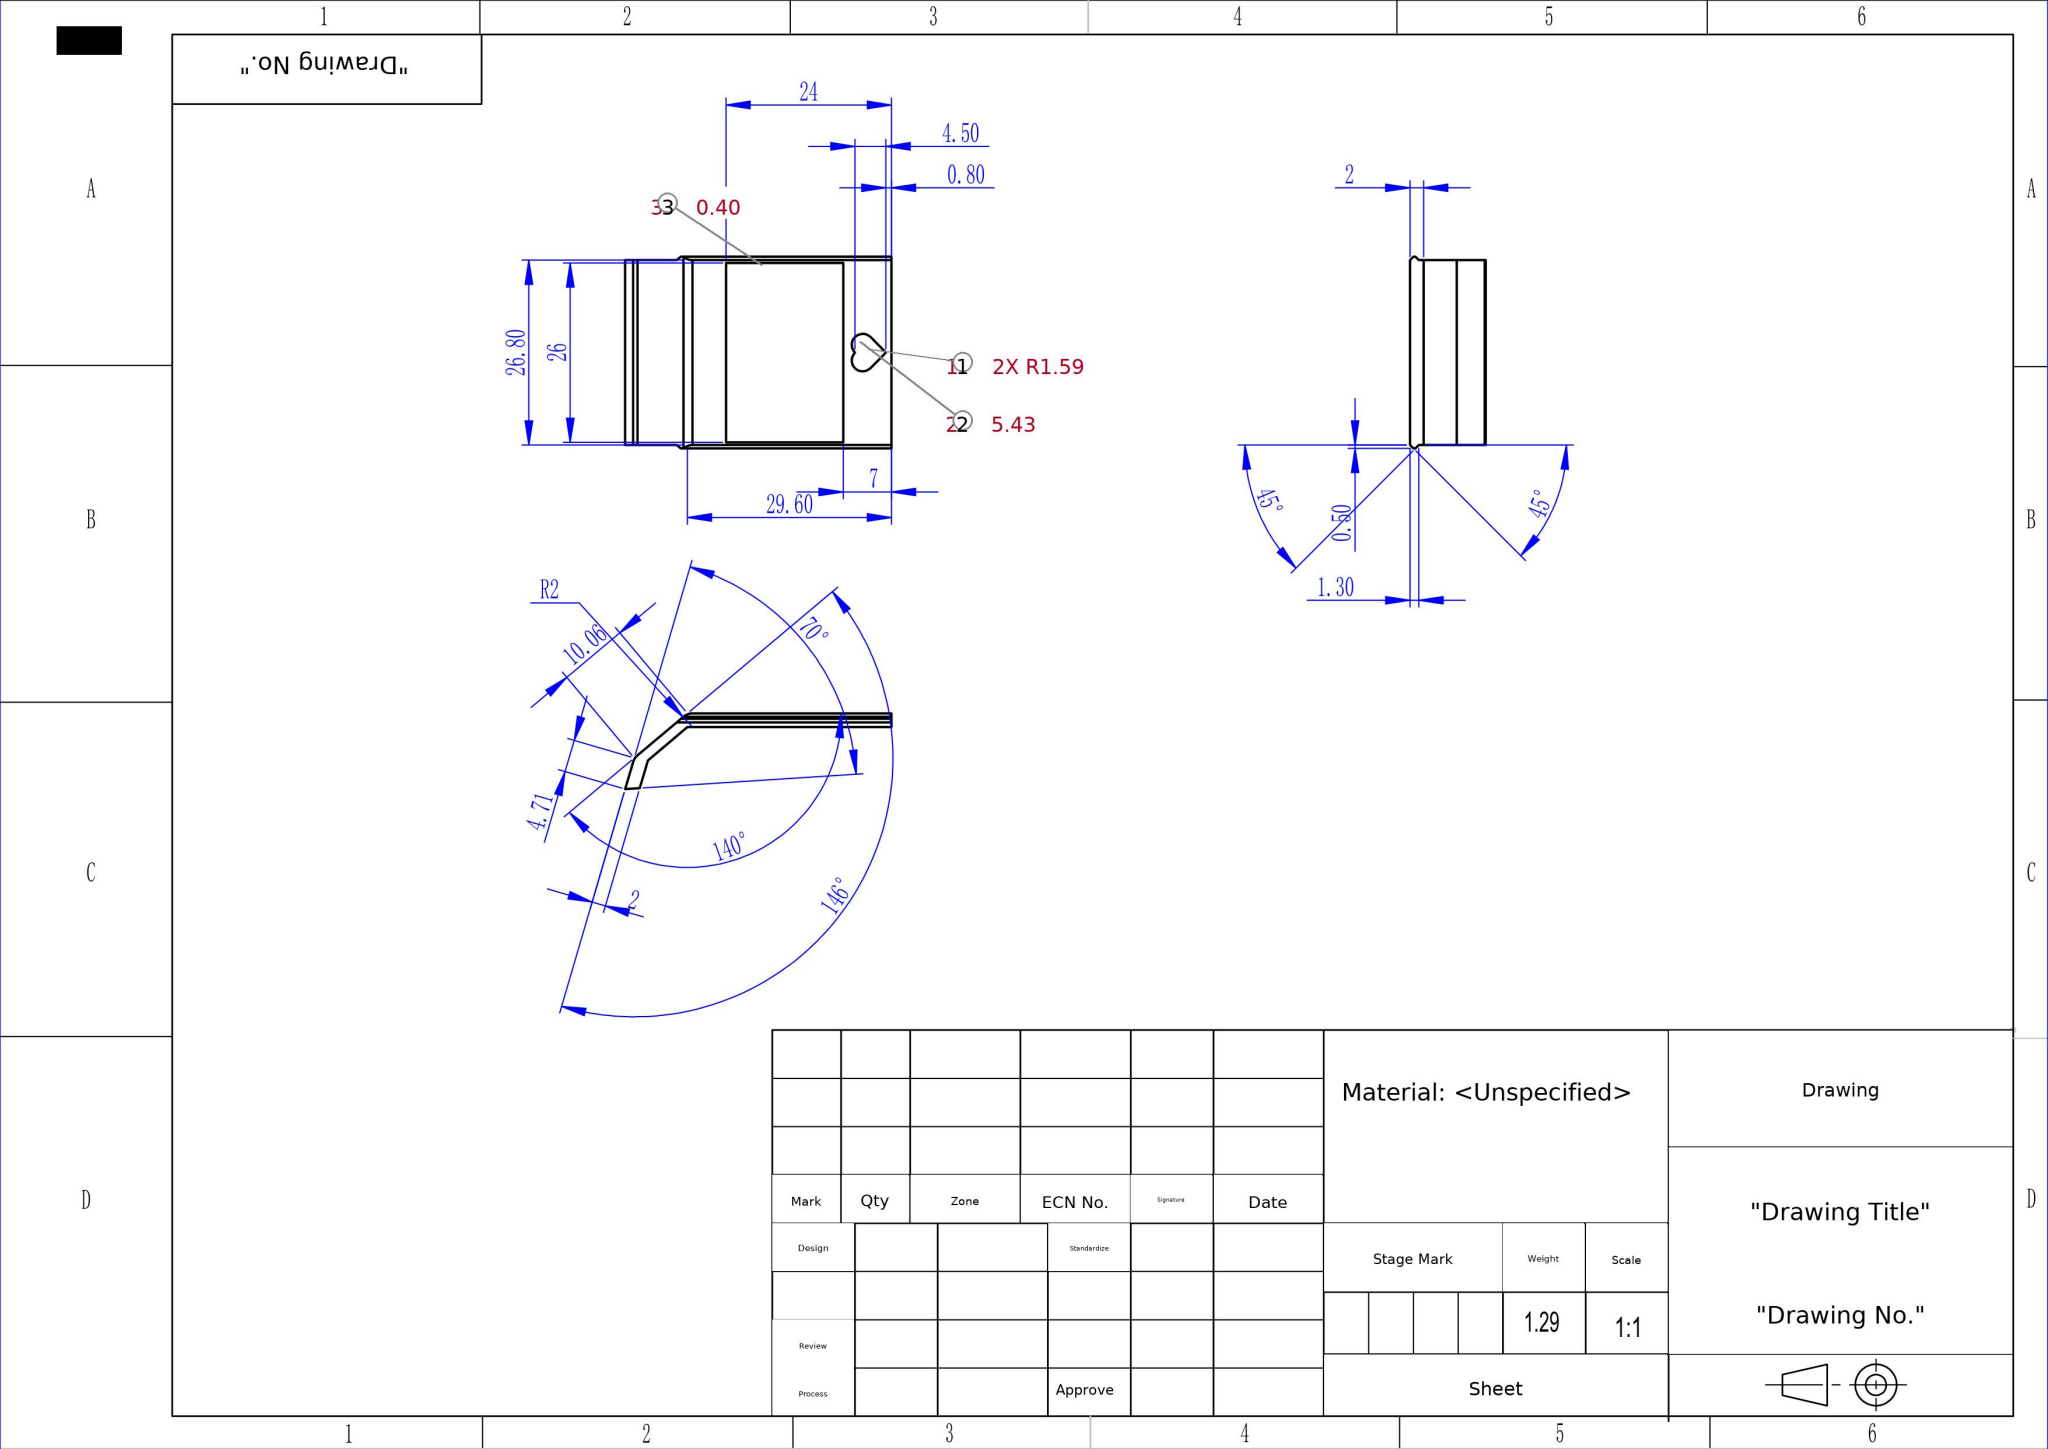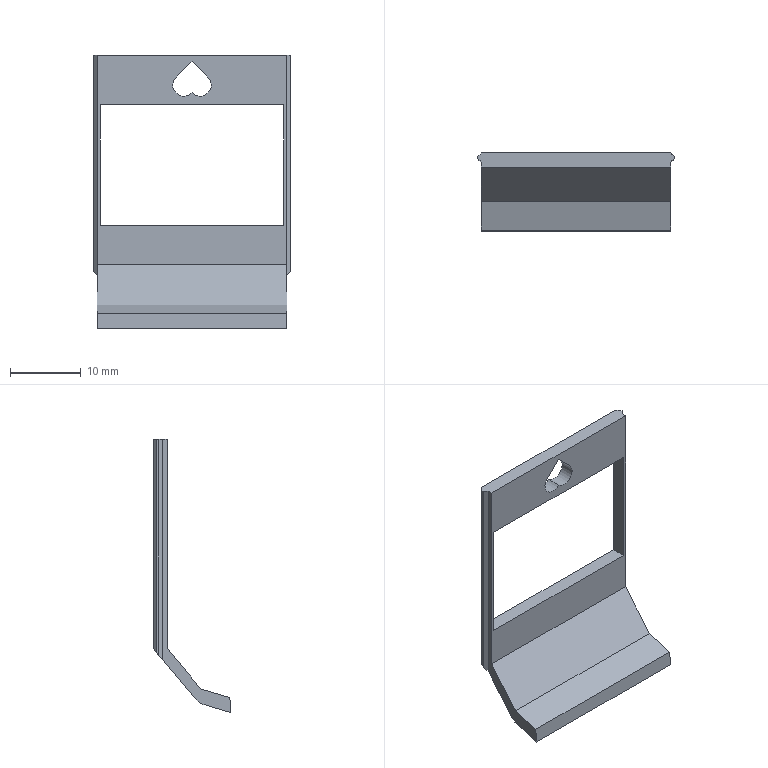Part | SolidWorks | mm | material <Unspecified> | 1 solid | 26 faces | box 27.8 x 10.99 x 38.63 mm | volume 1287 mm3 | plane 22 | cylinder 4 | commonest cylinder face diameters 4 x2 3.182 x2
build123d program:
from build123d import *

# Parameters (mm, degrees)
BOSS_EXTRUDE1_DEPTH = 2
BOSS_EXTRUDE2_DEPTH = 26.8
BOSS_EXTRUDE3_REACH = 49.867
FILLET1_R           = 2
CUT_EXTRUDE3_DEPTH  = 2


with BuildPart() as part:
    # Sketch1 → Boss-Extrude1 (new body)
    with BuildSketch(Plane(origin=(0, 0, 0), x_dir=(1, 0, 0), z_dir=(0, 1, 0))):
        Polygon((-26.8, 29.6), (0, 29.6), (0, 0), (-26.8, 0), align=None)
        Polygon((-26.4, 24), (-0.4, 24), (-0.4, 7), (-26.4, 7), align=None, mode=Mode.SUBTRACT)
    extrude(amount=BOSS_EXTRUDE1_DEPTH)

    # Sketch3 → Boss-Extrude2 (add)
    with BuildSketch(Plane(origin=(0, 0, 0), x_dir=(0, 0, -1), z_dir=(1, 0, 0))):
        Polygon((29.6, 2), (37.306, -4.466), (38.629, -8.987), (36.505, -8.85), (35.32, -4.8), (29.6, 0), align=None)
    extrude(amount=-BOSS_EXTRUDE2_DEPTH)

    # Boss-Extrude3: up to this plane
    boss_extrude3_end = Plane(origin=(-41.021, 2, -29.6), z_dir=(0, 0.766, -0.6428))
    # Sketch4 → Boss-Extrude3 (add, up to the surface)
    with BuildSketch(Plane.XY, mode=Mode.PRIVATE) as boss_extrude3_sk1:
        Polygon((-26.8, 2), (-27.3, 1.5), (-27.3, 1.2), (-26.8, 0.7), align=None)
    boss_extrude3_tool1 = split(extrude(boss_extrude3_sk1.sketch, amount=-BOSS_EXTRUDE3_REACH, mode=Mode.PRIVATE), bisect_by=boss_extrude3_end, keep=Keep.BOTH, mode=Mode.PRIVATE)
    add(boss_extrude3_tool1.solids().sort_by_distance((-26.998, 1.35, 0))[0])
    # Sketch4 → Boss-Extrude3 (add, up to the surface)
    with BuildSketch(Plane.XY, mode=Mode.PRIVATE) as boss_extrude3_sk2:
        Polygon((0, 0.7), (0, 2), (0.5, 1.5), (0.5, 1.2), align=None)
    boss_extrude3_tool2 = split(extrude(boss_extrude3_sk2.sketch, amount=-BOSS_EXTRUDE3_REACH, mode=Mode.PRIVATE), bisect_by=boss_extrude3_end, keep=Keep.BOTH, mode=Mode.PRIVATE)
    add(boss_extrude3_tool2.solids().sort_by_distance((0.1979, 1.35, 0))[0])

    # Fillet1
    fillet1_edges = [part.edges().sort_by_distance(p)[0] for p in [
        (-13.4, 2, -29.6),
        (-13.4, -4.466, -37.306),
    ]]
    fillet(fillet1_edges, radius=FILLET1_R)

    # Sketch8 → Cut-Extrude3 (cut)
    with BuildSketch(Plane(origin=(0, 2, 0), x_dir=(1, 0, 0), z_dir=(0, 1, 0))):
        with BuildLine():
            Line((-15.65, 3.05), (-13.4, 0.8))
            Line((-13.4, 0.8), (-11.15, 3.05))
            ThreePointArc((-11.15, 3.05), (-11.15, 5.3), (-13.4, 5.3))
            ThreePointArc((-13.4, 5.3), (-15.65, 5.3), (-15.65, 3.05))
        make_face()
    extrude(amount=-CUT_EXTRUDE3_DEPTH, mode=Mode.SUBTRACT)


solid = part.part